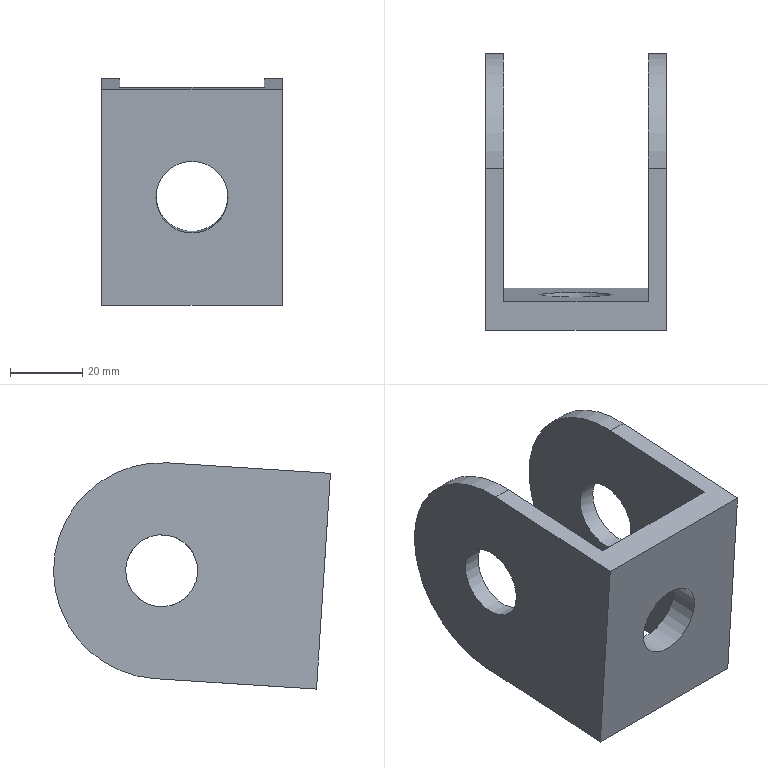Component | NX | CCJ-010 | 1 solid | 13 faces | box 50 x 76.84 x 62.84 mm | volume 54682 mm3 | plane 8 | cylinder 5 | commonest cylinder face diameters 20 x3 60 x2
STEP:
#1=CARTESIAN_POINT('',(0.,0.,0.));
#2=DIRECTION('',(0.,0.,1.));
#3=DIRECTION('',(1.,0.,0.));
#4=AXIS2_PLACEMENT_3D('',#1,#2,#3);
#5=CARTESIAN_POINT('',(5.,79.213,228.609));
#6=VERTEX_POINT('',#5);
#7=CARTESIAN_POINT('',(5.,42.29,226.225));
#8=VERTEX_POINT('',#7);
#9=CARTESIAN_POINT('',(5.,118.132,231.122));
#10=DIRECTION('',(0.,-0.9979,-0.06443));
#11=VECTOR('',#10,1.);
#12=LINE('',#9,#11);
#13=CARTESIAN_POINT('',(0.,109.151,230.542));
#14=DIRECTION('',(0.,0.06443,-0.9979));
#15=DIRECTION('',(-1.,0.,-0.));
#16=AXIS2_PLACEMENT_3D('',#13,#14,#15);
#17=PLANE('',#16);
#18=CARTESIAN_POINT('',(-5.,9.));
#19=DIRECTION('',(0.,-1.));
#20=VECTOR('',#19,1.);
#21=LINE('',#18,#20);
#22=(GEOMETRIC_REPRESENTATION_CONTEXT(2)PARAMETRIC_REPRESENTATION_CONTEXT()REPRESENTATION_CONTEXT('',''));
#23=DEFINITIONAL_REPRESENTATION('',(#21),#22);
#24=PCURVE('',#17,#23);
#25=CARTESIAN_POINT('',(5.,123.287,151.289));
#26=DIRECTION('',(-1.,0.,0.));
#27=DIRECTION('',(0.,0.9979,0.06443));
#28=AXIS2_PLACEMENT_3D('',#25,#26,#27);
#29=PLANE('',#28);
#30=CARTESIAN_POINT('',(-0.,-80.));
#31=DIRECTION('',(-1.,0.));
#32=VECTOR('',#31,1.);
#33=LINE('',#30,#32);
#34=(GEOMETRIC_REPRESENTATION_CONTEXT(2)PARAMETRIC_REPRESENTATION_CONTEXT()REPRESENTATION_CONTEXT('',''));
#35=DEFINITIONAL_REPRESENTATION('',(#33),#34);
#36=PCURVE('',#29,#35);
#37=SURFACE_CURVE('',#12,(#24,#36),.PCURVE_S1.);
#38=EDGE_CURVE('',#6,#8,#37,.T.);
#39=ORIENTED_EDGE('',*,*,#38,.F.);
#40=CARTESIAN_POINT('',(0.,79.213,228.609));
#41=VERTEX_POINT('',#40);
#42=CARTESIAN_POINT('',(0.,79.213,228.609));
#43=DIRECTION('',(-1.,0.,-0.));
#44=VECTOR('',#43,1.);
#45=LINE('',#42,#44);
#46=CARTESIAN_POINT('',(0.,-30.));
#47=DIRECTION('',(1.,0.));
#48=VECTOR('',#47,1.);
#49=LINE('',#46,#48);
#50=(GEOMETRIC_REPRESENTATION_CONTEXT(2)PARAMETRIC_REPRESENTATION_CONTEXT()REPRESENTATION_CONTEXT('',''));
#51=DEFINITIONAL_REPRESENTATION('',(#49),#50);
#52=PCURVE('',#17,#51);
#53=CARTESIAN_POINT('',(0.,81.146,198.672));
#54=DIRECTION('',(-1.,0.,-0.));
#55=DIRECTION('',(-0.,-0.06443,0.9979));
#56=AXIS2_PLACEMENT_3D('',#53,#54,#55);
#57=CYLINDRICAL_SURFACE('',#56,30.);
#58=CARTESIAN_POINT('',(0.,0.));
#59=DIRECTION('',(0.,1.));
#60=VECTOR('',#59,1.);
#61=LINE('',#58,#60);
#62=(GEOMETRIC_REPRESENTATION_CONTEXT(2)PARAMETRIC_REPRESENTATION_CONTEXT()REPRESENTATION_CONTEXT('',''));
#63=DEFINITIONAL_REPRESENTATION('',(#61),#62);
#64=PCURVE('',#57,#63);
#65=SURFACE_CURVE('',#45,(#52,#64),.PCURVE_S1.);
#66=EDGE_CURVE('',#6,#41,#65,.T.);
#67=ORIENTED_EDGE('',*,*,#66,.T.);
#68=CARTESIAN_POINT('',(0.,34.307,225.71));
#69=VERTEX_POINT('',#68);
#70=CARTESIAN_POINT('',(0.,109.151,230.542));
#71=DIRECTION('',(0.,-0.9979,-0.06443));
#72=VECTOR('',#71,1.);
#73=LINE('',#70,#72);
#74=CARTESIAN_POINT('',(0.,0.));
#75=DIRECTION('',(0.,-1.));
#76=VECTOR('',#75,1.);
#77=LINE('',#74,#76);
#78=(GEOMETRIC_REPRESENTATION_CONTEXT(2)PARAMETRIC_REPRESENTATION_CONTEXT()REPRESENTATION_CONTEXT('',''));
#79=DEFINITIONAL_REPRESENTATION('',(#77),#78);
#80=PCURVE('',#17,#79);
#81=CARTESIAN_POINT('',(0.,113.017,170.667));
#82=DIRECTION('',(1.,0.,0.));
#83=DIRECTION('',(0.,-0.9979,-0.06443));
#84=AXIS2_PLACEMENT_3D('',#81,#82,#83);
#85=PLANE('',#84);
#86=CARTESIAN_POINT('',(0.,-60.));
#87=DIRECTION('',(1.,0.));
#88=VECTOR('',#87,1.);
#89=LINE('',#86,#88);
#90=(GEOMETRIC_REPRESENTATION_CONTEXT(2)PARAMETRIC_REPRESENTATION_CONTEXT()REPRESENTATION_CONTEXT('',''));
#91=DEFINITIONAL_REPRESENTATION('',(#89),#90);
#92=PCURVE('',#85,#91);
#93=SURFACE_CURVE('',#73,(#80,#92),.PCURVE_S1.);
#94=EDGE_CURVE('',#41,#69,#93,.T.);
#95=ORIENTED_EDGE('',*,*,#94,.T.);
#96=CARTESIAN_POINT('',(50.,34.307,225.71));
#97=VERTEX_POINT('',#96);
#98=CARTESIAN_POINT('',(0.,34.307,225.71));
#99=DIRECTION('',(1.,-0.,0.));
#100=VECTOR('',#99,1.);
#101=LINE('',#98,#100);
#102=CARTESIAN_POINT('',(0.,-75.));
#103=DIRECTION('',(-1.,-0.));
#104=VECTOR('',#103,1.);
#105=LINE('',#102,#104);
#106=(GEOMETRIC_REPRESENTATION_CONTEXT(2)PARAMETRIC_REPRESENTATION_CONTEXT()REPRESENTATION_CONTEXT('',''));
#107=DEFINITIONAL_REPRESENTATION('',(#105),#106);
#108=PCURVE('',#17,#107);
#109=CARTESIAN_POINT('',(0.,34.307,225.71));
#110=DIRECTION('',(0.,0.9979,0.06443));
#111=DIRECTION('',(1.,0.,0.));
#112=AXIS2_PLACEMENT_3D('',#109,#110,#111);
#113=PLANE('',#112);
#114=CARTESIAN_POINT('',(0.,0.));
#115=DIRECTION('',(1.,-0.));
#116=VECTOR('',#115,1.);
#117=LINE('',#114,#116);
#118=(GEOMETRIC_REPRESENTATION_CONTEXT(2)PARAMETRIC_REPRESENTATION_CONTEXT()REPRESENTATION_CONTEXT('',''));
#119=DEFINITIONAL_REPRESENTATION('',(#117),#118);
#120=PCURVE('',#113,#119);
#121=SURFACE_CURVE('',#101,(#108,#120),.PCURVE_S1.);
#122=EDGE_CURVE('',#69,#97,#121,.T.);
#123=ORIENTED_EDGE('',*,*,#122,.T.);
#124=CARTESIAN_POINT('',(50.,79.213,228.609));
#125=VERTEX_POINT('',#124);
#126=CARTESIAN_POINT('',(50.,109.151,230.542));
#127=DIRECTION('',(0.,-0.9979,-0.06443));
#128=VECTOR('',#127,1.);
#129=LINE('',#126,#128);
#130=CARTESIAN_POINT('',(-50.,-0.));
#131=DIRECTION('',(0.,-1.));
#132=VECTOR('',#131,1.);
#133=LINE('',#130,#132);
#134=(GEOMETRIC_REPRESENTATION_CONTEXT(2)PARAMETRIC_REPRESENTATION_CONTEXT()REPRESENTATION_CONTEXT('',''));
#135=DEFINITIONAL_REPRESENTATION('',(#133),#134);
#136=PCURVE('',#17,#135);
#137=CARTESIAN_POINT('',(50.,109.151,230.542));
#138=DIRECTION('',(-1.,-0.,0.));
#139=DIRECTION('',(0.,-0.06443,0.9979));
#140=AXIS2_PLACEMENT_3D('',#137,#138,#139);
#141=PLANE('',#140);
#142=CARTESIAN_POINT('',(0.,0.));
#143=DIRECTION('',(0.,-1.));
#144=VECTOR('',#143,1.);
#145=LINE('',#142,#144);
#146=(GEOMETRIC_REPRESENTATION_CONTEXT(2)PARAMETRIC_REPRESENTATION_CONTEXT()REPRESENTATION_CONTEXT('',''));
#147=DEFINITIONAL_REPRESENTATION('',(#145),#146);
#148=PCURVE('',#141,#147);
#149=SURFACE_CURVE('',#129,(#136,#148),.PCURVE_S1.);
#150=EDGE_CURVE('',#125,#97,#149,.T.);
#151=ORIENTED_EDGE('',*,*,#150,.F.);
#152=CARTESIAN_POINT('',(45.,79.213,228.609));
#153=VERTEX_POINT('',#152);
#154=CARTESIAN_POINT('',(0.,79.213,228.609));
#155=DIRECTION('',(-1.,0.,-0.));
#156=VECTOR('',#155,1.);
#157=LINE('',#154,#156);
#158=CARTESIAN_POINT('',(0.,-30.));
#159=DIRECTION('',(1.,0.));
#160=VECTOR('',#159,1.);
#161=LINE('',#158,#160);
#162=(GEOMETRIC_REPRESENTATION_CONTEXT(2)PARAMETRIC_REPRESENTATION_CONTEXT()REPRESENTATION_CONTEXT('',''));
#163=DEFINITIONAL_REPRESENTATION('',(#161),#162);
#164=PCURVE('',#17,#163);
#165=CARTESIAN_POINT('',(0.,81.146,198.672));
#166=DIRECTION('',(-1.,0.,-0.));
#167=DIRECTION('',(-0.,-0.06443,0.9979));
#168=AXIS2_PLACEMENT_3D('',#165,#166,#167);
#169=CYLINDRICAL_SURFACE('',#168,30.);
#170=CARTESIAN_POINT('',(0.,0.));
#171=DIRECTION('',(0.,1.));
#172=VECTOR('',#171,1.);
#173=LINE('',#170,#172);
#174=(GEOMETRIC_REPRESENTATION_CONTEXT(2)PARAMETRIC_REPRESENTATION_CONTEXT()REPRESENTATION_CONTEXT('',''));
#175=DEFINITIONAL_REPRESENTATION('',(#173),#174);
#176=PCURVE('',#169,#175);
#177=SURFACE_CURVE('',#157,(#164,#176),.PCURVE_S1.);
#178=EDGE_CURVE('',#125,#153,#177,.T.);
#179=ORIENTED_EDGE('',*,*,#178,.T.);
#180=CARTESIAN_POINT('',(45.,42.29,226.225));
#181=VERTEX_POINT('',#180);
#182=CARTESIAN_POINT('',(45.,42.29,226.225));
#183=DIRECTION('',(0.,0.9979,0.06443));
#184=VECTOR('',#183,1.);
#185=LINE('',#182,#184);
#186=CARTESIAN_POINT('',(-45.,-67.));
#187=DIRECTION('',(-0.,1.));
#188=VECTOR('',#187,1.);
#189=LINE('',#186,#188);
#190=(GEOMETRIC_REPRESENTATION_CONTEXT(2)PARAMETRIC_REPRESENTATION_CONTEXT()REPRESENTATION_CONTEXT('',''));
#191=DEFINITIONAL_REPRESENTATION('',(#189),#190);
#192=PCURVE('',#17,#191);
#193=CARTESIAN_POINT('',(45.,47.445,146.392));
#194=DIRECTION('',(1.,0.,0.));
#195=DIRECTION('',(0.,-0.9979,-0.06443));
#196=AXIS2_PLACEMENT_3D('',#193,#194,#195);
#197=PLANE('',#196);
#198=CARTESIAN_POINT('',(-0.,-80.));
#199=DIRECTION('',(-1.,-0.));
#200=VECTOR('',#199,1.);
#201=LINE('',#198,#200);
#202=(GEOMETRIC_REPRESENTATION_CONTEXT(2)PARAMETRIC_REPRESENTATION_CONTEXT()REPRESENTATION_CONTEXT('',''));
#203=DEFINITIONAL_REPRESENTATION('',(#201),#202);
#204=PCURVE('',#197,#203);
#205=SURFACE_CURVE('',#185,(#192,#204),.PCURVE_S1.);
#206=EDGE_CURVE('',#181,#153,#205,.T.);
#207=ORIENTED_EDGE('',*,*,#206,.F.);
#208=CARTESIAN_POINT('',(5.,42.29,226.225));
#209=DIRECTION('',(1.,0.,0.));
#210=VECTOR('',#209,1.);
#211=LINE('',#208,#210);
#212=CARTESIAN_POINT('',(-5.,-67.));
#213=DIRECTION('',(-1.,-0.));
#214=VECTOR('',#213,1.);
#215=LINE('',#212,#214);
#216=(GEOMETRIC_REPRESENTATION_CONTEXT(2)PARAMETRIC_REPRESENTATION_CONTEXT()REPRESENTATION_CONTEXT('',''));
#217=DEFINITIONAL_REPRESENTATION('',(#215),#216);
#218=PCURVE('',#17,#217);
#219=CARTESIAN_POINT('',(5.,47.445,146.392));
#220=DIRECTION('',(0.,-0.9979,-0.06443));
#221=DIRECTION('',(-1.,0.,0.));
#222=AXIS2_PLACEMENT_3D('',#219,#220,#221);
#223=PLANE('',#222);
#224=CARTESIAN_POINT('',(0.,-80.));
#225=DIRECTION('',(-1.,0.));
#226=VECTOR('',#225,1.);
#227=LINE('',#224,#226);
#228=(GEOMETRIC_REPRESENTATION_CONTEXT(2)PARAMETRIC_REPRESENTATION_CONTEXT()REPRESENTATION_CONTEXT('',''));
#229=DEFINITIONAL_REPRESENTATION('',(#227),#228);
#230=PCURVE('',#223,#229);
#231=SURFACE_CURVE('',#211,(#218,#230),.PCURVE_S1.);
#232=EDGE_CURVE('',#8,#181,#231,.T.);
#233=ORIENTED_EDGE('',*,*,#232,.F.);
#234=EDGE_LOOP('',(#39,#67,#95,#123,#151,#179,#207,#233));
#235=FACE_BOUND('',#234,.T.);
#236=ADVANCED_FACE('',(#235),#17,.F.);
#237=CARTESIAN_POINT('',(5.,83.079,168.734));
#238=VERTEX_POINT('',#237);
#239=CARTESIAN_POINT('',(5.,81.146,198.672));
#240=DIRECTION('',(1.,0.,0.));
#241=DIRECTION('',(0.,0.9979,0.06443));
#242=AXIS2_PLACEMENT_3D('',#239,#240,#241);
#243=CIRCLE('',#242,30.);
#244=CARTESIAN_POINT('',(7.854,-5.));
#245=DIRECTION('',(-1.,-0.));
#246=VECTOR('',#245,1.);
#247=LINE('',#244,#246);
#248=(GEOMETRIC_REPRESENTATION_CONTEXT(2)PARAMETRIC_REPRESENTATION_CONTEXT()REPRESENTATION_CONTEXT('',''));
#249=DEFINITIONAL_REPRESENTATION('',(#247),#248);
#250=PCURVE('',#57,#249);
#251=CARTESIAN_POINT('',(-9.,-50.));
#252=CARTESIAN_POINT('',(-9.,-101.962));
#253=CARTESIAN_POINT('',(-54.,-75.981));
#254=CARTESIAN_POINT('',(-99.,-50.));
#255=CARTESIAN_POINT('',(-54.,-24.019));
#256=CARTESIAN_POINT('',(-9.,1.962));
#257=CARTESIAN_POINT('',(-9.,-50.));
#258=(BOUNDED_CURVE()B_SPLINE_CURVE(2,(#251,#252,#253,#254,#255,#256,#257),.UNSPECIFIED.,.T.,.F.)B_SPLINE_CURVE_WITH_KNOTS((1,2,2,2,2,1),(-2.094,0.,2.094,4.189,6.283,8.378),.UNSPECIFIED.)CURVE()GEOMETRIC_REPRESENTATION_ITEM()RATIONAL_B_SPLINE_CURVE((1.,0.5,1.,0.5,1.,0.5,1.))REPRESENTATION_ITEM(''));
#259=(GEOMETRIC_REPRESENTATION_CONTEXT(2)PARAMETRIC_REPRESENTATION_CONTEXT()REPRESENTATION_CONTEXT('',''));
#260=DEFINITIONAL_REPRESENTATION('',(#258),#259);
#261=PCURVE('',#29,#260);
#262=SURFACE_CURVE('',#243,(#250,#261),.PCURVE_S1.);
#263=EDGE_CURVE('',#238,#6,#262,.T.);
#264=ORIENTED_EDGE('',*,*,#263,.F.);
#265=CARTESIAN_POINT('',(0.,83.079,168.734));
#266=VERTEX_POINT('',#265);
#267=CARTESIAN_POINT('',(50.,83.079,168.734));
#268=DIRECTION('',(1.,0.,0.));
#269=VECTOR('',#268,1.);
#270=LINE('',#267,#269);
#271=CARTESIAN_POINT('',(3.142,-50.));
#272=DIRECTION('',(0.,-1.));
#273=VECTOR('',#272,1.);
#274=LINE('',#271,#273);
#275=(GEOMETRIC_REPRESENTATION_CONTEXT(2)PARAMETRIC_REPRESENTATION_CONTEXT()REPRESENTATION_CONTEXT('',''));
#276=DEFINITIONAL_REPRESENTATION('',(#274),#275);
#277=PCURVE('',#57,#276);
#278=CARTESIAN_POINT('',(50.,113.017,170.667));
#279=DIRECTION('',(0.,-0.06443,0.9979));
#280=DIRECTION('',(0.,-0.9979,-0.06443));
#281=AXIS2_PLACEMENT_3D('',#278,#279,#280);
#282=PLANE('',#281);
#283=CARTESIAN_POINT('',(30.,0.));
#284=DIRECTION('',(0.,1.));
#285=VECTOR('',#284,1.);
#286=LINE('',#283,#285);
#287=(GEOMETRIC_REPRESENTATION_CONTEXT(2)PARAMETRIC_REPRESENTATION_CONTEXT()REPRESENTATION_CONTEXT('',''));
#288=DEFINITIONAL_REPRESENTATION('',(#286),#287);
#289=PCURVE('',#282,#288);
#290=SURFACE_CURVE('',#270,(#277,#289),.PCURVE_S1.);
#291=EDGE_CURVE('',#266,#238,#290,.T.);
#292=ORIENTED_EDGE('',*,*,#291,.F.);
#293=CARTESIAN_POINT('',(0.,81.146,198.672));
#294=DIRECTION('',(-1.,0.,0.));
#295=DIRECTION('',(0.,-0.9979,-0.06443));
#296=AXIS2_PLACEMENT_3D('',#293,#294,#295);
#297=CIRCLE('',#296,30.);
#298=CARTESIAN_POINT('',(-1.571,-0.));
#299=DIRECTION('',(1.,0.));
#300=VECTOR('',#299,1.);
#301=LINE('',#298,#300);
#302=(GEOMETRIC_REPRESENTATION_CONTEXT(2)PARAMETRIC_REPRESENTATION_CONTEXT()REPRESENTATION_CONTEXT('',''));
#303=DEFINITIONAL_REPRESENTATION('',(#301),#302);
#304=PCURVE('',#57,#303);
#305=CARTESIAN_POINT('',(60.,-30.));
#306=CARTESIAN_POINT('',(60.,-81.962));
#307=CARTESIAN_POINT('',(15.,-55.981));
#308=CARTESIAN_POINT('',(-30.,-30.));
#309=CARTESIAN_POINT('',(15.,-4.019));
#310=CARTESIAN_POINT('',(60.,21.962));
#311=CARTESIAN_POINT('',(60.,-30.));
#312=(BOUNDED_CURVE()B_SPLINE_CURVE(2,(#305,#306,#307,#308,#309,#310,#311),.UNSPECIFIED.,.T.,.F.)B_SPLINE_CURVE_WITH_KNOTS((1,2,2,2,2,1),(-2.094,0.,2.094,4.189,6.283,8.378),.UNSPECIFIED.)CURVE()GEOMETRIC_REPRESENTATION_ITEM()RATIONAL_B_SPLINE_CURVE((1.,0.5,1.,0.5,1.,0.5,1.))REPRESENTATION_ITEM(''));
#313=(GEOMETRIC_REPRESENTATION_CONTEXT(2)PARAMETRIC_REPRESENTATION_CONTEXT()REPRESENTATION_CONTEXT('',''));
#314=DEFINITIONAL_REPRESENTATION('',(#312),#313);
#315=PCURVE('',#85,#314);
#316=SURFACE_CURVE('',#297,(#304,#315),.PCURVE_S1.);
#317=EDGE_CURVE('',#41,#266,#316,.T.);
#318=ORIENTED_EDGE('',*,*,#317,.F.);
#319=ORIENTED_EDGE('',*,*,#66,.F.);
#320=EDGE_LOOP('',(#264,#292,#318,#319));
#321=FACE_BOUND('',#320,.T.);
#322=ADVANCED_FACE('',(#321),#57,.T.);
#323=CARTESIAN_POINT('',(5.,71.167,198.027));
#324=VERTEX_POINT('',#323);
#325=CARTESIAN_POINT('',(5.,91.126,199.316));
#326=VERTEX_POINT('',#325);
#327=CARTESIAN_POINT('',(5.,81.146,198.672));
#328=DIRECTION('',(1.,0.,0.));
#329=DIRECTION('',(0.,0.9979,0.06443));
#330=AXIS2_PLACEMENT_3D('',#327,#328,#329);
#331=CIRCLE('',#330,10.);
#332=CARTESIAN_POINT('',(-10.,81.146,198.672));
#333=DIRECTION('',(1.,0.,0.));
#334=DIRECTION('',(0.,-0.9979,-0.06443));
#335=AXIS2_PLACEMENT_3D('',#332,#333,#334);
#336=CYLINDRICAL_SURFACE('',#335,10.);
#337=CARTESIAN_POINT('',(-3.142,15.));
#338=DIRECTION('',(1.,0.));
#339=VECTOR('',#338,1.);
#340=LINE('',#337,#339);
#341=(GEOMETRIC_REPRESENTATION_CONTEXT(2)PARAMETRIC_REPRESENTATION_CONTEXT()REPRESENTATION_CONTEXT('',''));
#342=DEFINITIONAL_REPRESENTATION('',(#340),#341);
#343=PCURVE('',#336,#342);
#344=CARTESIAN_POINT('',(-29.,-50.));
#345=CARTESIAN_POINT('',(-29.,-67.321));
#346=CARTESIAN_POINT('',(-44.,-58.66));
#347=CARTESIAN_POINT('',(-59.,-50.));
#348=CARTESIAN_POINT('',(-44.,-41.34));
#349=CARTESIAN_POINT('',(-29.,-32.679));
#350=CARTESIAN_POINT('',(-29.,-50.));
#351=(BOUNDED_CURVE()B_SPLINE_CURVE(2,(#344,#345,#346,#347,#348,#349,#350),.UNSPECIFIED.,.T.,.F.)B_SPLINE_CURVE_WITH_KNOTS((1,2,2,2,2,1),(-2.094,0.,2.094,4.189,6.283,8.378),.UNSPECIFIED.)CURVE()GEOMETRIC_REPRESENTATION_ITEM()RATIONAL_B_SPLINE_CURVE((1.,0.5,1.,0.5,1.,0.5,1.))REPRESENTATION_ITEM(''));
#352=(GEOMETRIC_REPRESENTATION_CONTEXT(2)PARAMETRIC_REPRESENTATION_CONTEXT()REPRESENTATION_CONTEXT('',''));
#353=DEFINITIONAL_REPRESENTATION('',(#351),#352);
#354=PCURVE('',#29,#353);
#355=SURFACE_CURVE('',#331,(#343,#354),.PCURVE_S1.);
#356=EDGE_CURVE('',#324,#326,#355,.T.);
#357=ORIENTED_EDGE('',*,*,#356,.F.);
#358=CARTESIAN_POINT('',(0.,71.167,198.027));
#359=VERTEX_POINT('',#358);
#360=CARTESIAN_POINT('',(0.,71.167,198.027));
#361=CARTESIAN_POINT('',(5.,71.167,198.027));
#362=B_SPLINE_CURVE_WITH_KNOTS('',1,(#360,#361),.UNSPECIFIED.,.F.,.F.,(2,2),(10.,15.),.PIECEWISE_BEZIER_KNOTS.);
#363=CARTESIAN_POINT('',(0.,0.));
#364=DIRECTION('',(0.,1.));
#365=VECTOR('',#364,1.);
#366=LINE('',#363,#365);
#367=(GEOMETRIC_REPRESENTATION_CONTEXT(2)PARAMETRIC_REPRESENTATION_CONTEXT()REPRESENTATION_CONTEXT('',''));
#368=DEFINITIONAL_REPRESENTATION('',(#366),#367);
#369=PCURVE('',#336,#368);
#370=CARTESIAN_POINT('',(6.283,0.));
#371=DIRECTION('',(0.,1.));
#372=VECTOR('',#371,1.);
#373=LINE('',#370,#372);
#374=(GEOMETRIC_REPRESENTATION_CONTEXT(2)PARAMETRIC_REPRESENTATION_CONTEXT()REPRESENTATION_CONTEXT('',''));
#375=DEFINITIONAL_REPRESENTATION('',(#373),#374);
#376=PCURVE('',#336,#375);
#377=SEAM_CURVE('',#362,(#369,#376),.PCURVE_S1.);
#378=EDGE_CURVE('',#359,#324,#377,.T.);
#379=ORIENTED_EDGE('',*,*,#378,.F.);
#380=CARTESIAN_POINT('',(0.,81.146,198.672));
#381=DIRECTION('',(1.,0.,0.));
#382=DIRECTION('',(0.,-0.9979,-0.06443));
#383=AXIS2_PLACEMENT_3D('',#380,#381,#382);
#384=CIRCLE('',#383,10.);
#385=CARTESIAN_POINT('',(0.,10.));
#386=DIRECTION('',(1.,0.));
#387=VECTOR('',#386,1.);
#388=LINE('',#385,#387);
#389=(GEOMETRIC_REPRESENTATION_CONTEXT(2)PARAMETRIC_REPRESENTATION_CONTEXT()REPRESENTATION_CONTEXT('',''));
#390=DEFINITIONAL_REPRESENTATION('',(#388),#389);
#391=PCURVE('',#336,#390);
#392=CARTESIAN_POINT('',(30.,-30.));
#393=DIRECTION('',(1.,0.));
#394=AXIS2_PLACEMENT_2D('',#392,#393);
#395=CIRCLE('',#394,10.);
#396=(GEOMETRIC_REPRESENTATION_CONTEXT(2)PARAMETRIC_REPRESENTATION_CONTEXT()REPRESENTATION_CONTEXT('',''));
#397=DEFINITIONAL_REPRESENTATION('',(#395),#396);
#398=PCURVE('',#85,#397);
#399=SURFACE_CURVE('',#384,(#391,#398),.PCURVE_S1.);
#400=EDGE_CURVE('',#359,#359,#399,.T.);
#401=ORIENTED_EDGE('',*,*,#400,.T.);
#402=ORIENTED_EDGE('',*,*,#378,.T.);
#403=CARTESIAN_POINT('',(5.,81.146,198.672));
#404=DIRECTION('',(1.,0.,0.));
#405=DIRECTION('',(0.,0.9979,0.06443));
#406=AXIS2_PLACEMENT_3D('',#403,#404,#405);
#407=CIRCLE('',#406,10.);
#408=CARTESIAN_POINT('',(3.142,15.));
#409=DIRECTION('',(1.,0.));
#410=VECTOR('',#409,1.);
#411=LINE('',#408,#410);
#412=(GEOMETRIC_REPRESENTATION_CONTEXT(2)PARAMETRIC_REPRESENTATION_CONTEXT()REPRESENTATION_CONTEXT('',''));
#413=DEFINITIONAL_REPRESENTATION('',(#411),#412);
#414=PCURVE('',#336,#413);
#415=CARTESIAN_POINT('',(-29.,-50.));
#416=CARTESIAN_POINT('',(-29.,-67.321));
#417=CARTESIAN_POINT('',(-44.,-58.66));
#418=CARTESIAN_POINT('',(-59.,-50.));
#419=CARTESIAN_POINT('',(-44.,-41.34));
#420=CARTESIAN_POINT('',(-29.,-32.679));
#421=CARTESIAN_POINT('',(-29.,-50.));
#422=(BOUNDED_CURVE()B_SPLINE_CURVE(2,(#415,#416,#417,#418,#419,#420,#421),.UNSPECIFIED.,.T.,.F.)B_SPLINE_CURVE_WITH_KNOTS((1,2,2,2,2,1),(-2.094,0.,2.094,4.189,6.283,8.378),.UNSPECIFIED.)CURVE()GEOMETRIC_REPRESENTATION_ITEM()RATIONAL_B_SPLINE_CURVE((1.,0.5,1.,0.5,1.,0.5,1.))REPRESENTATION_ITEM(''));
#423=(GEOMETRIC_REPRESENTATION_CONTEXT(2)PARAMETRIC_REPRESENTATION_CONTEXT()REPRESENTATION_CONTEXT('',''));
#424=DEFINITIONAL_REPRESENTATION('',(#422),#423);
#425=PCURVE('',#29,#424);
#426=SURFACE_CURVE('',#407,(#414,#425),.PCURVE_S1.);
#427=EDGE_CURVE('',#326,#324,#426,.T.);
#428=ORIENTED_EDGE('',*,*,#427,.F.);
#429=EDGE_LOOP('',(#357,#379,#401,#402,#428));
#430=FACE_BOUND('',#429,.F.);
#431=ADVANCED_FACE('',(#430),#336,.F.);
#432=CARTESIAN_POINT('',(45.,71.167,198.027));
#433=VERTEX_POINT('',#432);
#434=CARTESIAN_POINT('',(45.,81.146,198.672));
#435=DIRECTION('',(-1.,0.,0.));
#436=DIRECTION('',(0.,-0.9979,-0.06443));
#437=AXIS2_PLACEMENT_3D('',#434,#435,#436);
#438=CIRCLE('',#437,10.);
#439=CARTESIAN_POINT('',(-10.,81.146,198.672));
#440=DIRECTION('',(1.,0.,0.));
#441=DIRECTION('',(0.,-0.9979,-0.06443));
#442=AXIS2_PLACEMENT_3D('',#439,#440,#441);
#443=CYLINDRICAL_SURFACE('',#442,10.);
#444=CARTESIAN_POINT('',(6.283,55.));
#445=DIRECTION('',(-1.,0.));
#446=VECTOR('',#445,1.);
#447=LINE('',#444,#446);
#448=(GEOMETRIC_REPRESENTATION_CONTEXT(2)PARAMETRIC_REPRESENTATION_CONTEXT()REPRESENTATION_CONTEXT('',''));
#449=DEFINITIONAL_REPRESENTATION('',(#447),#448);
#450=PCURVE('',#443,#449);
#451=CARTESIAN_POINT('',(-27.,-50.));
#452=CARTESIAN_POINT('',(-27.,-67.321));
#453=CARTESIAN_POINT('',(-42.,-58.66));
#454=CARTESIAN_POINT('',(-57.,-50.));
#455=CARTESIAN_POINT('',(-42.,-41.34));
#456=CARTESIAN_POINT('',(-27.,-32.679));
#457=CARTESIAN_POINT('',(-27.,-50.));
#458=(BOUNDED_CURVE()B_SPLINE_CURVE(2,(#451,#452,#453,#454,#455,#456,#457),.UNSPECIFIED.,.T.,.F.)B_SPLINE_CURVE_WITH_KNOTS((1,2,2,2,2,1),(-2.094,0.,2.094,4.189,6.283,8.378),.UNSPECIFIED.)CURVE()GEOMETRIC_REPRESENTATION_ITEM()RATIONAL_B_SPLINE_CURVE((1.,0.5,1.,0.5,1.,0.5,1.))REPRESENTATION_ITEM(''));
#459=(GEOMETRIC_REPRESENTATION_CONTEXT(2)PARAMETRIC_REPRESENTATION_CONTEXT()REPRESENTATION_CONTEXT('',''));
#460=DEFINITIONAL_REPRESENTATION('',(#458),#459);
#461=PCURVE('',#197,#460);
#462=SURFACE_CURVE('',#438,(#450,#461),.PCURVE_S1.);
#463=EDGE_CURVE('',#433,#433,#462,.T.);
#464=ORIENTED_EDGE('',*,*,#463,.F.);
#465=CARTESIAN_POINT('',(50.,71.167,198.027));
#466=VERTEX_POINT('',#465);
#467=CARTESIAN_POINT('',(45.,71.167,198.027));
#468=CARTESIAN_POINT('',(50.,71.167,198.027));
#469=B_SPLINE_CURVE_WITH_KNOTS('',1,(#467,#468),.UNSPECIFIED.,.F.,.F.,(2,2),(55.,60.),.PIECEWISE_BEZIER_KNOTS.);
#470=CARTESIAN_POINT('',(6.283,0.));
#471=DIRECTION('',(0.,1.));
#472=VECTOR('',#471,1.);
#473=LINE('',#470,#472);
#474=(GEOMETRIC_REPRESENTATION_CONTEXT(2)PARAMETRIC_REPRESENTATION_CONTEXT()REPRESENTATION_CONTEXT('',''));
#475=DEFINITIONAL_REPRESENTATION('',(#473),#474);
#476=PCURVE('',#443,#475);
#477=CARTESIAN_POINT('',(0.,0.));
#478=DIRECTION('',(0.,1.));
#479=VECTOR('',#478,1.);
#480=LINE('',#477,#479);
#481=(GEOMETRIC_REPRESENTATION_CONTEXT(2)PARAMETRIC_REPRESENTATION_CONTEXT()REPRESENTATION_CONTEXT('',''));
#482=DEFINITIONAL_REPRESENTATION('',(#480),#481);
#483=PCURVE('',#443,#482);
#484=SEAM_CURVE('',#469,(#476,#483),.PCURVE_S1.);
#485=EDGE_CURVE('',#433,#466,#484,.T.);
#486=ORIENTED_EDGE('',*,*,#485,.T.);
#487=CARTESIAN_POINT('',(50.,81.791,188.693));
#488=VERTEX_POINT('',#487);
#489=CARTESIAN_POINT('',(50.,81.146,198.672));
#490=DIRECTION('',(1.,0.,0.));
#491=DIRECTION('',(0.,0.06443,-0.9979));
#492=AXIS2_PLACEMENT_3D('',#489,#490,#491);
#493=CIRCLE('',#492,10.);
#494=CARTESIAN_POINT('',(1.571,60.));
#495=DIRECTION('',(1.,0.));
#496=VECTOR('',#495,1.);
#497=LINE('',#494,#496);
#498=(GEOMETRIC_REPRESENTATION_CONTEXT(2)PARAMETRIC_REPRESENTATION_CONTEXT()REPRESENTATION_CONTEXT('',''));
#499=DEFINITIONAL_REPRESENTATION('',(#497),#498);
#500=PCURVE('',#443,#499);
#501=CARTESIAN_POINT('',(-40.,-30.));
#502=CARTESIAN_POINT('',(-40.,-12.679));
#503=CARTESIAN_POINT('',(-25.,-21.34));
#504=CARTESIAN_POINT('',(-10.,-30.));
#505=CARTESIAN_POINT('',(-25.,-38.66));
#506=CARTESIAN_POINT('',(-40.,-47.321));
#507=CARTESIAN_POINT('',(-40.,-30.));
#508=(BOUNDED_CURVE()B_SPLINE_CURVE(2,(#501,#502,#503,#504,#505,#506,#507),.UNSPECIFIED.,.T.,.F.)B_SPLINE_CURVE_WITH_KNOTS((1,2,2,2,2,1),(-2.094,0.,2.094,4.189,6.283,8.378),.UNSPECIFIED.)CURVE()GEOMETRIC_REPRESENTATION_ITEM()RATIONAL_B_SPLINE_CURVE((1.,0.5,1.,0.5,1.,0.5,1.))REPRESENTATION_ITEM(''));
#509=(GEOMETRIC_REPRESENTATION_CONTEXT(2)PARAMETRIC_REPRESENTATION_CONTEXT()REPRESENTATION_CONTEXT('',''));
#510=DEFINITIONAL_REPRESENTATION('',(#508),#509);
#511=PCURVE('',#141,#510);
#512=SURFACE_CURVE('',#493,(#500,#511),.PCURVE_S1.);
#513=EDGE_CURVE('',#488,#466,#512,.T.);
#514=ORIENTED_EDGE('',*,*,#513,.F.);
#515=CARTESIAN_POINT('',(50.,81.146,198.672));
#516=DIRECTION('',(1.,0.,0.));
#517=DIRECTION('',(0.,0.06443,-0.9979));
#518=AXIS2_PLACEMENT_3D('',#515,#516,#517);
#519=CIRCLE('',#518,10.);
#520=CARTESIAN_POINT('',(-4.712,60.));
#521=DIRECTION('',(1.,0.));
#522=VECTOR('',#521,1.);
#523=LINE('',#520,#522);
#524=(GEOMETRIC_REPRESENTATION_CONTEXT(2)PARAMETRIC_REPRESENTATION_CONTEXT()REPRESENTATION_CONTEXT('',''));
#525=DEFINITIONAL_REPRESENTATION('',(#523),#524);
#526=PCURVE('',#443,#525);
#527=CARTESIAN_POINT('',(-40.,-30.));
#528=CARTESIAN_POINT('',(-40.,-12.679));
#529=CARTESIAN_POINT('',(-25.,-21.34));
#530=CARTESIAN_POINT('',(-10.,-30.));
#531=CARTESIAN_POINT('',(-25.,-38.66));
#532=CARTESIAN_POINT('',(-40.,-47.321));
#533=CARTESIAN_POINT('',(-40.,-30.));
#534=(BOUNDED_CURVE()B_SPLINE_CURVE(2,(#527,#528,#529,#530,#531,#532,#533),.UNSPECIFIED.,.T.,.F.)B_SPLINE_CURVE_WITH_KNOTS((1,2,2,2,2,1),(-2.094,0.,2.094,4.189,6.283,8.378),.UNSPECIFIED.)CURVE()GEOMETRIC_REPRESENTATION_ITEM()RATIONAL_B_SPLINE_CURVE((1.,0.5,1.,0.5,1.,0.5,1.))REPRESENTATION_ITEM(''));
#535=(GEOMETRIC_REPRESENTATION_CONTEXT(2)PARAMETRIC_REPRESENTATION_CONTEXT()REPRESENTATION_CONTEXT('',''));
#536=DEFINITIONAL_REPRESENTATION('',(#534),#535);
#537=PCURVE('',#141,#536);
#538=SURFACE_CURVE('',#519,(#526,#537),.PCURVE_S1.);
#539=EDGE_CURVE('',#466,#488,#538,.T.);
#540=ORIENTED_EDGE('',*,*,#539,.F.);
#541=ORIENTED_EDGE('',*,*,#485,.F.);
#542=EDGE_LOOP('',(#464,#486,#514,#540,#541));
#543=FACE_BOUND('',#542,.F.);
#544=ADVANCED_FACE('',(#543),#443,.F.);
#545=CARTESIAN_POINT('',(50.,83.079,168.734));
#546=VERTEX_POINT('',#545);
#547=CARTESIAN_POINT('',(50.,38.173,165.835));
#548=VERTEX_POINT('',#547);
#549=CARTESIAN_POINT('',(50.,113.017,170.667));
#550=DIRECTION('',(0.,-0.9979,-0.06443));
#551=VECTOR('',#550,1.);
#552=LINE('',#549,#551);
#553=CARTESIAN_POINT('',(-60.,0.));
#554=DIRECTION('',(0.,-1.));
#555=VECTOR('',#554,1.);
#556=LINE('',#553,#555);
#557=(GEOMETRIC_REPRESENTATION_CONTEXT(2)PARAMETRIC_REPRESENTATION_CONTEXT()REPRESENTATION_CONTEXT('',''));
#558=DEFINITIONAL_REPRESENTATION('',(#556),#557);
#559=PCURVE('',#141,#558);
#560=CARTESIAN_POINT('',(0.,0.));
#561=DIRECTION('',(1.,0.));
#562=VECTOR('',#561,1.);
#563=LINE('',#560,#562);
#564=(GEOMETRIC_REPRESENTATION_CONTEXT(2)PARAMETRIC_REPRESENTATION_CONTEXT()REPRESENTATION_CONTEXT('',''));
#565=DEFINITIONAL_REPRESENTATION('',(#563),#564);
#566=PCURVE('',#282,#565);
#567=SURFACE_CURVE('',#552,(#559,#566),.PCURVE_S1.);
#568=EDGE_CURVE('',#546,#548,#567,.T.);
#569=ORIENTED_EDGE('',*,*,#568,.F.);
#570=CARTESIAN_POINT('',(50.,81.146,198.672));
#571=DIRECTION('',(1.,0.,-0.));
#572=DIRECTION('',(0.,-0.06443,0.9979));
#573=AXIS2_PLACEMENT_3D('',#570,#571,#572);
#574=CIRCLE('',#573,30.);
#575=CARTESIAN_POINT('',(0.,-30.));
#576=CARTESIAN_POINT('',(0.,-81.962));
#577=CARTESIAN_POINT('',(-45.,-55.981));
#578=CARTESIAN_POINT('',(-90.,-30.));
#579=CARTESIAN_POINT('',(-45.,-4.019));
#580=CARTESIAN_POINT('',(0.,21.962));
#581=CARTESIAN_POINT('',(0.,-30.));
#582=(BOUNDED_CURVE()B_SPLINE_CURVE(2,(#575,#576,#577,#578,#579,#580,#581),.UNSPECIFIED.,.T.,.F.)B_SPLINE_CURVE_WITH_KNOTS((1,2,2,2,2,1),(-2.094,0.,2.094,4.189,6.283,8.378),.UNSPECIFIED.)CURVE()GEOMETRIC_REPRESENTATION_ITEM()RATIONAL_B_SPLINE_CURVE((1.,0.5,1.,0.5,1.,0.5,1.))REPRESENTATION_ITEM(''));
#583=(GEOMETRIC_REPRESENTATION_CONTEXT(2)PARAMETRIC_REPRESENTATION_CONTEXT()REPRESENTATION_CONTEXT('',''));
#584=DEFINITIONAL_REPRESENTATION('',(#582),#583);
#585=PCURVE('',#141,#584);
#586=CARTESIAN_POINT('',(6.283,-50.));
#587=DIRECTION('',(-1.,-0.));
#588=VECTOR('',#587,1.);
#589=LINE('',#586,#588);
#590=(GEOMETRIC_REPRESENTATION_CONTEXT(2)PARAMETRIC_REPRESENTATION_CONTEXT()REPRESENTATION_CONTEXT('',''));
#591=DEFINITIONAL_REPRESENTATION('',(#589),#590);
#592=PCURVE('',#169,#591);
#593=SURFACE_CURVE('',#574,(#585,#592),.PCURVE_S1.);
#594=EDGE_CURVE('',#546,#125,#593,.T.);
#595=ORIENTED_EDGE('',*,*,#594,.T.);
#596=ORIENTED_EDGE('',*,*,#150,.T.);
#597=CARTESIAN_POINT('',(50.,34.307,225.71));
#598=DIRECTION('',(-0.,0.06443,-0.9979));
#599=VECTOR('',#598,1.);
#600=LINE('',#597,#599);
#601=CARTESIAN_POINT('',(0.,-75.));
#602=DIRECTION('',(-1.,0.));
#603=VECTOR('',#602,1.);
#604=LINE('',#601,#603);
#605=(GEOMETRIC_REPRESENTATION_CONTEXT(2)PARAMETRIC_REPRESENTATION_CONTEXT()REPRESENTATION_CONTEXT('',''));
#606=DEFINITIONAL_REPRESENTATION('',(#604),#605);
#607=PCURVE('',#141,#606);
#608=CARTESIAN_POINT('',(50.,0.));
#609=DIRECTION('',(-0.,1.));
#610=VECTOR('',#609,1.);
#611=LINE('',#608,#610);
#612=(GEOMETRIC_REPRESENTATION_CONTEXT(2)PARAMETRIC_REPRESENTATION_CONTEXT()REPRESENTATION_CONTEXT('',''));
#613=DEFINITIONAL_REPRESENTATION('',(#611),#612);
#614=PCURVE('',#113,#613);
#615=SURFACE_CURVE('',#600,(#607,#614),.PCURVE_S1.);
#616=EDGE_CURVE('',#97,#548,#615,.T.);
#617=ORIENTED_EDGE('',*,*,#616,.T.);
#618=EDGE_LOOP('',(#569,#595,#596,#617));
#619=FACE_BOUND('',#618,.T.);
#620=ORIENTED_EDGE('',*,*,#513,.F.);
#621=ORIENTED_EDGE('',*,*,#539,.F.);
#622=EDGE_LOOP('',(#620,#621));
#623=FACE_BOUND('',#622,.T.);
#624=ADVANCED_FACE('',(#619,#623),#141,.F.);
#625=ORIENTED_EDGE('',*,*,#400,.T.);
#626=EDGE_LOOP('',(#625));
#627=FACE_BOUND('',#626,.T.);
#628=ORIENTED_EDGE('',*,*,#317,.T.);
#629=CARTESIAN_POINT('',(0.,38.173,165.835));
#630=VERTEX_POINT('',#629);
#631=CARTESIAN_POINT('',(0.,113.017,170.667));
#632=DIRECTION('',(0.,-0.9979,-0.06443));
#633=VECTOR('',#632,1.);
#634=LINE('',#631,#633);
#635=CARTESIAN_POINT('',(0.,0.));
#636=DIRECTION('',(1.,0.));
#637=VECTOR('',#636,1.);
#638=LINE('',#635,#637);
#639=(GEOMETRIC_REPRESENTATION_CONTEXT(2)PARAMETRIC_REPRESENTATION_CONTEXT()REPRESENTATION_CONTEXT('',''));
#640=DEFINITIONAL_REPRESENTATION('',(#638),#639);
#641=PCURVE('',#85,#640);
#642=CARTESIAN_POINT('',(0.,-50.));
#643=DIRECTION('',(1.,0.));
#644=VECTOR('',#643,1.);
#645=LINE('',#642,#644);
#646=(GEOMETRIC_REPRESENTATION_CONTEXT(2)PARAMETRIC_REPRESENTATION_CONTEXT()REPRESENTATION_CONTEXT('',''));
#647=DEFINITIONAL_REPRESENTATION('',(#645),#646);
#648=PCURVE('',#282,#647);
#649=SURFACE_CURVE('',#634,(#641,#648),.PCURVE_S1.);
#650=EDGE_CURVE('',#266,#630,#649,.T.);
#651=ORIENTED_EDGE('',*,*,#650,.T.);
#652=CARTESIAN_POINT('',(0.,38.173,165.835));
#653=DIRECTION('',(0.,-0.06443,0.9979));
#654=VECTOR('',#653,1.);
#655=LINE('',#652,#654);
#656=CARTESIAN_POINT('',(75.,-0.));
#657=DIRECTION('',(0.,-1.));
#658=VECTOR('',#657,1.);
#659=LINE('',#656,#658);
#660=(GEOMETRIC_REPRESENTATION_CONTEXT(2)PARAMETRIC_REPRESENTATION_CONTEXT()REPRESENTATION_CONTEXT('',''));
#661=DEFINITIONAL_REPRESENTATION('',(#659),#660);
#662=PCURVE('',#85,#661);
#663=CARTESIAN_POINT('',(0.,60.));
#664=DIRECTION('',(0.,-1.));
#665=VECTOR('',#664,1.);
#666=LINE('',#663,#665);
#667=(GEOMETRIC_REPRESENTATION_CONTEXT(2)PARAMETRIC_REPRESENTATION_CONTEXT()REPRESENTATION_CONTEXT('',''));
#668=DEFINITIONAL_REPRESENTATION('',(#666),#667);
#669=PCURVE('',#113,#668);
#670=SURFACE_CURVE('',#655,(#662,#669),.PCURVE_S1.);
#671=EDGE_CURVE('',#630,#69,#670,.T.);
#672=ORIENTED_EDGE('',*,*,#671,.T.);
#673=ORIENTED_EDGE('',*,*,#94,.F.);
#674=EDGE_LOOP('',(#628,#651,#672,#673));
#675=FACE_BOUND('',#674,.T.);
#676=ADVANCED_FACE('',(#627,#675),#85,.F.);
#677=ORIENTED_EDGE('',*,*,#291,.T.);
#678=CARTESIAN_POINT('',(5.,46.156,166.35));
#679=VERTEX_POINT('',#678);
#680=CARTESIAN_POINT('',(5.,113.017,170.667));
#681=DIRECTION('',(0.,-0.9979,-0.06443));
#682=VECTOR('',#681,1.);
#683=LINE('',#680,#682);
#684=CARTESIAN_POINT('',(0.,-45.));
#685=DIRECTION('',(1.,0.));
#686=VECTOR('',#685,1.);
#687=LINE('',#684,#686);
#688=(GEOMETRIC_REPRESENTATION_CONTEXT(2)PARAMETRIC_REPRESENTATION_CONTEXT()REPRESENTATION_CONTEXT('',''));
#689=DEFINITIONAL_REPRESENTATION('',(#687),#688);
#690=PCURVE('',#282,#689);
#691=CARTESIAN_POINT('',(-9.,-20.));
#692=DIRECTION('',(-1.,0.));
#693=VECTOR('',#692,1.);
#694=LINE('',#691,#693);
#695=(GEOMETRIC_REPRESENTATION_CONTEXT(2)PARAMETRIC_REPRESENTATION_CONTEXT()REPRESENTATION_CONTEXT('',''));
#696=DEFINITIONAL_REPRESENTATION('',(#694),#695);
#697=PCURVE('',#29,#696);
#698=SURFACE_CURVE('',#683,(#690,#697),.PCURVE_S1.);
#699=EDGE_CURVE('',#238,#679,#698,.T.);
#700=ORIENTED_EDGE('',*,*,#699,.T.);
#701=CARTESIAN_POINT('',(45.,46.156,166.35));
#702=VERTEX_POINT('',#701);
#703=CARTESIAN_POINT('',(50.,46.156,166.35));
#704=DIRECTION('',(1.,0.,0.));
#705=VECTOR('',#704,1.);
#706=LINE('',#703,#705);
#707=CARTESIAN_POINT('',(67.,0.));
#708=DIRECTION('',(0.,1.));
#709=VECTOR('',#708,1.);
#710=LINE('',#707,#709);
#711=(GEOMETRIC_REPRESENTATION_CONTEXT(2)PARAMETRIC_REPRESENTATION_CONTEXT()REPRESENTATION_CONTEXT('',''));
#712=DEFINITIONAL_REPRESENTATION('',(#710),#711);
#713=PCURVE('',#282,#712);
#714=CARTESIAN_POINT('',(-45.,-20.));
#715=DIRECTION('',(-1.,0.));
#716=VECTOR('',#715,1.);
#717=LINE('',#714,#716);
#718=(GEOMETRIC_REPRESENTATION_CONTEXT(2)PARAMETRIC_REPRESENTATION_CONTEXT()REPRESENTATION_CONTEXT('',''));
#719=DEFINITIONAL_REPRESENTATION('',(#717),#718);
#720=PCURVE('',#223,#719);
#721=SURFACE_CURVE('',#706,(#713,#720),.PCURVE_S1.);
#722=EDGE_CURVE('',#679,#702,#721,.T.);
#723=ORIENTED_EDGE('',*,*,#722,.T.);
#724=CARTESIAN_POINT('',(45.,83.079,168.734));
#725=VERTEX_POINT('',#724);
#726=CARTESIAN_POINT('',(45.,113.017,170.667));
#727=DIRECTION('',(0.,0.9979,0.06443));
#728=VECTOR('',#727,1.);
#729=LINE('',#726,#728);
#730=CARTESIAN_POINT('',(0.,-5.));
#731=DIRECTION('',(-1.,0.));
#732=VECTOR('',#731,1.);
#733=LINE('',#730,#732);
#734=(GEOMETRIC_REPRESENTATION_CONTEXT(2)PARAMETRIC_REPRESENTATION_CONTEXT()REPRESENTATION_CONTEXT('',''));
#735=DEFINITIONAL_REPRESENTATION('',(#733),#734);
#736=PCURVE('',#282,#735);
#737=CARTESIAN_POINT('',(-67.,-20.));
#738=DIRECTION('',(-1.,0.));
#739=VECTOR('',#738,1.);
#740=LINE('',#737,#739);
#741=(GEOMETRIC_REPRESENTATION_CONTEXT(2)PARAMETRIC_REPRESENTATION_CONTEXT()REPRESENTATION_CONTEXT('',''));
#742=DEFINITIONAL_REPRESENTATION('',(#740),#741);
#743=PCURVE('',#197,#742);
#744=SURFACE_CURVE('',#729,(#736,#743),.PCURVE_S1.);
#745=EDGE_CURVE('',#702,#725,#744,.T.);
#746=ORIENTED_EDGE('',*,*,#745,.T.);
#747=CARTESIAN_POINT('',(50.,83.079,168.734));
#748=DIRECTION('',(1.,0.,0.));
#749=VECTOR('',#748,1.);
#750=LINE('',#747,#749);
#751=CARTESIAN_POINT('',(30.,0.));
#752=DIRECTION('',(0.,1.));
#753=VECTOR('',#752,1.);
#754=LINE('',#751,#753);
#755=(GEOMETRIC_REPRESENTATION_CONTEXT(2)PARAMETRIC_REPRESENTATION_CONTEXT()REPRESENTATION_CONTEXT('',''));
#756=DEFINITIONAL_REPRESENTATION('',(#754),#755);
#757=PCURVE('',#282,#756);
#758=CARTESIAN_POINT('',(3.142,-50.));
#759=DIRECTION('',(0.,-1.));
#760=VECTOR('',#759,1.);
#761=LINE('',#758,#760);
#762=(GEOMETRIC_REPRESENTATION_CONTEXT(2)PARAMETRIC_REPRESENTATION_CONTEXT()REPRESENTATION_CONTEXT('',''));
#763=DEFINITIONAL_REPRESENTATION('',(#761),#762);
#764=PCURVE('',#169,#763);
#765=SURFACE_CURVE('',#750,(#757,#764),.PCURVE_S1.);
#766=EDGE_CURVE('',#725,#546,#765,.T.);
#767=ORIENTED_EDGE('',*,*,#766,.T.);
#768=ORIENTED_EDGE('',*,*,#568,.T.);
#769=CARTESIAN_POINT('',(50.,38.173,165.835));
#770=DIRECTION('',(-1.,0.,0.));
#771=VECTOR('',#770,1.);
#772=LINE('',#769,#771);
#773=CARTESIAN_POINT('',(75.,0.));
#774=DIRECTION('',(0.,-1.));
#775=VECTOR('',#774,1.);
#776=LINE('',#773,#775);
#777=(GEOMETRIC_REPRESENTATION_CONTEXT(2)PARAMETRIC_REPRESENTATION_CONTEXT()REPRESENTATION_CONTEXT('',''));
#778=DEFINITIONAL_REPRESENTATION('',(#776),#777);
#779=PCURVE('',#282,#778);
#780=CARTESIAN_POINT('',(50.,60.));
#781=DIRECTION('',(-1.,0.));
#782=VECTOR('',#781,1.);
#783=LINE('',#780,#782);
#784=(GEOMETRIC_REPRESENTATION_CONTEXT(2)PARAMETRIC_REPRESENTATION_CONTEXT()REPRESENTATION_CONTEXT('',''));
#785=DEFINITIONAL_REPRESENTATION('',(#783),#784);
#786=PCURVE('',#113,#785);
#787=SURFACE_CURVE('',#772,(#779,#786),.PCURVE_S1.);
#788=EDGE_CURVE('',#548,#630,#787,.T.);
#789=ORIENTED_EDGE('',*,*,#788,.T.);
#790=ORIENTED_EDGE('',*,*,#650,.F.);
#791=EDGE_LOOP('',(#677,#700,#723,#746,#767,#768,#789,#790));
#792=FACE_BOUND('',#791,.T.);
#793=ADVANCED_FACE('',(#792),#282,.F.);
#794=CARTESIAN_POINT('',(35.,36.24,195.772));
#795=VERTEX_POINT('',#794);
#796=CARTESIAN_POINT('',(15.,36.24,195.772));
#797=VERTEX_POINT('',#796);
#798=CARTESIAN_POINT('',(25.,36.24,195.772));
#799=DIRECTION('',(0.,0.9979,0.06443));
#800=DIRECTION('',(1.,0.,0.));
#801=AXIS2_PLACEMENT_3D('',#798,#799,#800);
#802=CIRCLE('',#801,10.);
#803=CARTESIAN_POINT('',(25.,30.));
#804=DIRECTION('',(1.,0.));
#805=AXIS2_PLACEMENT_2D('',#803,#804);
#806=CIRCLE('',#805,10.);
#807=(GEOMETRIC_REPRESENTATION_CONTEXT(2)PARAMETRIC_REPRESENTATION_CONTEXT()REPRESENTATION_CONTEXT('',''));
#808=DEFINITIONAL_REPRESENTATION('',(#806),#807);
#809=PCURVE('',#113,#808);
#810=CARTESIAN_POINT('',(25.,96.115,199.638));
#811=DIRECTION('',(0.,-0.9979,-0.06443));
#812=DIRECTION('',(-1.,0.,0.));
#813=AXIS2_PLACEMENT_3D('',#810,#811,#812);
#814=CYLINDRICAL_SURFACE('',#813,10.);
#815=CARTESIAN_POINT('',(3.142,60.));
#816=DIRECTION('',(-1.,0.));
#817=VECTOR('',#816,1.);
#818=LINE('',#815,#817);
#819=(GEOMETRIC_REPRESENTATION_CONTEXT(2)PARAMETRIC_REPRESENTATION_CONTEXT()REPRESENTATION_CONTEXT('',''));
#820=DEFINITIONAL_REPRESENTATION('',(#818),#819);
#821=PCURVE('',#814,#820);
#822=SURFACE_CURVE('',#802,(#809,#821),.PCURVE_S1.);
#823=EDGE_CURVE('',#795,#797,#822,.T.);
#824=ORIENTED_EDGE('',*,*,#823,.T.);
#825=CARTESIAN_POINT('',(25.,36.24,195.772));
#826=DIRECTION('',(0.,0.9979,0.06443));
#827=DIRECTION('',(1.,0.,0.));
#828=AXIS2_PLACEMENT_3D('',#825,#826,#827);
#829=CIRCLE('',#828,10.);
#830=CARTESIAN_POINT('',(25.,30.));
#831=DIRECTION('',(1.,0.));
#832=AXIS2_PLACEMENT_2D('',#830,#831);
#833=CIRCLE('',#832,10.);
#834=(GEOMETRIC_REPRESENTATION_CONTEXT(2)PARAMETRIC_REPRESENTATION_CONTEXT()REPRESENTATION_CONTEXT('',''));
#835=DEFINITIONAL_REPRESENTATION('',(#833),#834);
#836=PCURVE('',#113,#835);
#837=CARTESIAN_POINT('',(9.425,60.));
#838=DIRECTION('',(-1.,0.));
#839=VECTOR('',#838,1.);
#840=LINE('',#837,#839);
#841=(GEOMETRIC_REPRESENTATION_CONTEXT(2)PARAMETRIC_REPRESENTATION_CONTEXT()REPRESENTATION_CONTEXT('',''));
#842=DEFINITIONAL_REPRESENTATION('',(#840),#841);
#843=PCURVE('',#814,#842);
#844=SURFACE_CURVE('',#829,(#836,#843),.PCURVE_S1.);
#845=EDGE_CURVE('',#797,#795,#844,.T.);
#846=ORIENTED_EDGE('',*,*,#845,.T.);
#847=EDGE_LOOP('',(#824,#846));
#848=FACE_BOUND('',#847,.T.);
#849=ORIENTED_EDGE('',*,*,#671,.F.);
#850=ORIENTED_EDGE('',*,*,#788,.F.);
#851=ORIENTED_EDGE('',*,*,#616,.F.);
#852=ORIENTED_EDGE('',*,*,#122,.F.);
#853=EDGE_LOOP('',(#849,#850,#851,#852));
#854=FACE_BOUND('',#853,.T.);
#855=ADVANCED_FACE('',(#848,#854),#113,.F.);
#856=CARTESIAN_POINT('',(15.,44.223,196.288));
#857=VERTEX_POINT('',#856);
#858=CARTESIAN_POINT('',(25.,44.223,196.288));
#859=DIRECTION('',(0.,-0.9979,-0.06443));
#860=DIRECTION('',(-1.,0.,0.));
#861=AXIS2_PLACEMENT_3D('',#858,#859,#860);
#862=CIRCLE('',#861,10.);
#863=CARTESIAN_POINT('',(0.,52.));
#864=DIRECTION('',(1.,0.));
#865=VECTOR('',#864,1.);
#866=LINE('',#863,#865);
#867=(GEOMETRIC_REPRESENTATION_CONTEXT(2)PARAMETRIC_REPRESENTATION_CONTEXT()REPRESENTATION_CONTEXT('',''));
#868=DEFINITIONAL_REPRESENTATION('',(#866),#867);
#869=PCURVE('',#814,#868);
#870=CARTESIAN_POINT('',(-20.,-50.));
#871=DIRECTION('',(1.,0.));
#872=AXIS2_PLACEMENT_2D('',#870,#871);
#873=CIRCLE('',#872,10.);
#874=(GEOMETRIC_REPRESENTATION_CONTEXT(2)PARAMETRIC_REPRESENTATION_CONTEXT()REPRESENTATION_CONTEXT('',''));
#875=DEFINITIONAL_REPRESENTATION('',(#873),#874);
#876=PCURVE('',#223,#875);
#877=SURFACE_CURVE('',#862,(#869,#876),.PCURVE_S1.);
#878=EDGE_CURVE('',#857,#857,#877,.T.);
#879=ORIENTED_EDGE('',*,*,#878,.T.);
#880=CARTESIAN_POINT('',(15.,44.223,196.288));
#881=CARTESIAN_POINT('',(15.,36.24,195.772));
#882=B_SPLINE_CURVE_WITH_KNOTS('',1,(#880,#881),.UNSPECIFIED.,.F.,.F.,(2,2),(52.,60.),.PIECEWISE_BEZIER_KNOTS.);
#883=CARTESIAN_POINT('',(6.283,0.));
#884=DIRECTION('',(0.,1.));
#885=VECTOR('',#884,1.);
#886=LINE('',#883,#885);
#887=(GEOMETRIC_REPRESENTATION_CONTEXT(2)PARAMETRIC_REPRESENTATION_CONTEXT()REPRESENTATION_CONTEXT('',''));
#888=DEFINITIONAL_REPRESENTATION('',(#886),#887);
#889=PCURVE('',#814,#888);
#890=CARTESIAN_POINT('',(0.,0.));
#891=DIRECTION('',(0.,1.));
#892=VECTOR('',#891,1.);
#893=LINE('',#890,#892);
#894=(GEOMETRIC_REPRESENTATION_CONTEXT(2)PARAMETRIC_REPRESENTATION_CONTEXT()REPRESENTATION_CONTEXT('',''));
#895=DEFINITIONAL_REPRESENTATION('',(#893),#894);
#896=PCURVE('',#814,#895);
#897=SEAM_CURVE('',#882,(#889,#896),.PCURVE_S1.);
#898=EDGE_CURVE('',#857,#797,#897,.T.);
#899=ORIENTED_EDGE('',*,*,#898,.T.);
#900=ORIENTED_EDGE('',*,*,#845,.T.);
#901=ORIENTED_EDGE('',*,*,#823,.T.);
#902=ORIENTED_EDGE('',*,*,#898,.F.);
#903=EDGE_LOOP('',(#879,#899,#900,#901,#902));
#904=FACE_BOUND('',#903,.F.);
#905=ADVANCED_FACE('',(#904),#814,.F.);
#906=CARTESIAN_POINT('',(45.,81.146,198.672));
#907=DIRECTION('',(-1.,0.,0.));
#908=DIRECTION('',(0.,-0.9979,-0.06443));
#909=AXIS2_PLACEMENT_3D('',#906,#907,#908);
#910=CIRCLE('',#909,30.);
#911=CARTESIAN_POINT('',(-1.571,-45.));
#912=DIRECTION('',(1.,0.));
#913=VECTOR('',#912,1.);
#914=LINE('',#911,#913);
#915=(GEOMETRIC_REPRESENTATION_CONTEXT(2)PARAMETRIC_REPRESENTATION_CONTEXT()REPRESENTATION_CONTEXT('',''));
#916=DEFINITIONAL_REPRESENTATION('',(#914),#915);
#917=PCURVE('',#169,#916);
#918=CARTESIAN_POINT('',(-7.,-50.));
#919=CARTESIAN_POINT('',(-7.,-101.962));
#920=CARTESIAN_POINT('',(-52.,-75.981));
#921=CARTESIAN_POINT('',(-97.,-50.));
#922=CARTESIAN_POINT('',(-52.,-24.019));
#923=CARTESIAN_POINT('',(-7.,1.962));
#924=CARTESIAN_POINT('',(-7.,-50.));
#925=(BOUNDED_CURVE()B_SPLINE_CURVE(2,(#918,#919,#920,#921,#922,#923,#924),.UNSPECIFIED.,.T.,.F.)B_SPLINE_CURVE_WITH_KNOTS((1,2,2,2,2,1),(-2.094,0.,2.094,4.189,6.283,8.378),.UNSPECIFIED.)CURVE()GEOMETRIC_REPRESENTATION_ITEM()RATIONAL_B_SPLINE_CURVE((1.,0.5,1.,0.5,1.,0.5,1.))REPRESENTATION_ITEM(''));
#926=(GEOMETRIC_REPRESENTATION_CONTEXT(2)PARAMETRIC_REPRESENTATION_CONTEXT()REPRESENTATION_CONTEXT('',''));
#927=DEFINITIONAL_REPRESENTATION('',(#925),#926);
#928=PCURVE('',#197,#927);
#929=SURFACE_CURVE('',#910,(#917,#928),.PCURVE_S1.);
#930=EDGE_CURVE('',#153,#725,#929,.T.);
#931=ORIENTED_EDGE('',*,*,#930,.F.);
#932=ORIENTED_EDGE('',*,*,#178,.F.);
#933=ORIENTED_EDGE('',*,*,#594,.F.);
#934=ORIENTED_EDGE('',*,*,#766,.F.);
#935=EDGE_LOOP('',(#931,#932,#933,#934));
#936=FACE_BOUND('',#935,.T.);
#937=ADVANCED_FACE('',(#936),#169,.T.);
#938=ORIENTED_EDGE('',*,*,#878,.T.);
#939=EDGE_LOOP('',(#938));
#940=FACE_BOUND('',#939,.T.);
#941=CARTESIAN_POINT('',(5.,47.445,146.392));
#942=DIRECTION('',(0.,0.06443,-0.9979));
#943=VECTOR('',#942,1.);
#944=LINE('',#941,#943);
#945=CARTESIAN_POINT('',(0.,0.));
#946=DIRECTION('',(0.,1.));
#947=VECTOR('',#946,1.);
#948=LINE('',#945,#947);
#949=(GEOMETRIC_REPRESENTATION_CONTEXT(2)PARAMETRIC_REPRESENTATION_CONTEXT()REPRESENTATION_CONTEXT('',''));
#950=DEFINITIONAL_REPRESENTATION('',(#948),#949);
#951=PCURVE('',#223,#950);
#952=CARTESIAN_POINT('',(-76.,0.));
#953=DIRECTION('',(0.,1.));
#954=VECTOR('',#953,1.);
#955=LINE('',#952,#954);
#956=(GEOMETRIC_REPRESENTATION_CONTEXT(2)PARAMETRIC_REPRESENTATION_CONTEXT()REPRESENTATION_CONTEXT('',''));
#957=DEFINITIONAL_REPRESENTATION('',(#955),#956);
#958=PCURVE('',#29,#957);
#959=SURFACE_CURVE('',#944,(#951,#958),.PCURVE_S1.);
#960=EDGE_CURVE('',#8,#679,#959,.T.);
#961=ORIENTED_EDGE('',*,*,#960,.F.);
#962=ORIENTED_EDGE('',*,*,#232,.T.);
#963=CARTESIAN_POINT('',(45.,47.445,146.392));
#964=DIRECTION('',(0.,0.06443,-0.9979));
#965=VECTOR('',#964,1.);
#966=LINE('',#963,#965);
#967=CARTESIAN_POINT('',(-40.,0.));
#968=DIRECTION('',(0.,1.));
#969=VECTOR('',#968,1.);
#970=LINE('',#967,#969);
#971=(GEOMETRIC_REPRESENTATION_CONTEXT(2)PARAMETRIC_REPRESENTATION_CONTEXT()REPRESENTATION_CONTEXT('',''));
#972=DEFINITIONAL_REPRESENTATION('',(#970),#971);
#973=PCURVE('',#223,#972);
#974=CARTESIAN_POINT('',(0.,0.));
#975=DIRECTION('',(0.,1.));
#976=VECTOR('',#975,1.);
#977=LINE('',#974,#976);
#978=(GEOMETRIC_REPRESENTATION_CONTEXT(2)PARAMETRIC_REPRESENTATION_CONTEXT()REPRESENTATION_CONTEXT('',''));
#979=DEFINITIONAL_REPRESENTATION('',(#977),#978);
#980=PCURVE('',#197,#979);
#981=SURFACE_CURVE('',#966,(#973,#980),.PCURVE_S1.);
#982=EDGE_CURVE('',#181,#702,#981,.T.);
#983=ORIENTED_EDGE('',*,*,#982,.T.);
#984=ORIENTED_EDGE('',*,*,#722,.F.);
#985=EDGE_LOOP('',(#961,#962,#983,#984));
#986=FACE_BOUND('',#985,.T.);
#987=ADVANCED_FACE('',(#940,#986),#223,.F.);
#988=ORIENTED_EDGE('',*,*,#263,.T.);
#989=ORIENTED_EDGE('',*,*,#38,.T.);
#990=ORIENTED_EDGE('',*,*,#960,.T.);
#991=ORIENTED_EDGE('',*,*,#699,.F.);
#992=EDGE_LOOP('',(#988,#989,#990,#991));
#993=FACE_BOUND('',#992,.T.);
#994=ORIENTED_EDGE('',*,*,#427,.F.);
#995=ORIENTED_EDGE('',*,*,#356,.F.);
#996=EDGE_LOOP('',(#994,#995));
#997=FACE_BOUND('',#996,.T.);
#998=ADVANCED_FACE('',(#993,#997),#29,.F.);
#999=ORIENTED_EDGE('',*,*,#982,.F.);
#1000=ORIENTED_EDGE('',*,*,#206,.T.);
#1001=ORIENTED_EDGE('',*,*,#930,.T.);
#1002=ORIENTED_EDGE('',*,*,#745,.F.);
#1003=EDGE_LOOP('',(#999,#1000,#1001,#1002));
#1004=FACE_BOUND('',#1003,.T.);
#1005=ORIENTED_EDGE('',*,*,#463,.F.);
#1006=EDGE_LOOP('',(#1005));
#1007=FACE_BOUND('',#1006,.T.);
#1008=ADVANCED_FACE('',(#1004,#1007),#197,.F.);
#1009=CLOSED_SHELL('',(#236,#322,#431,#544,#624,#676,#793,#855,#905,#937,#987,#998,#1008));
#1010=MANIFOLD_SOLID_BREP('',#1009);
#1011=(LENGTH_UNIT()NAMED_UNIT(*)SI_UNIT(.MILLI.,.METRE.));
#1012=UNCERTAINTY_MEASURE_WITH_UNIT(LENGTH_MEASURE(0.000002),#1011,'','');
#1013=(NAMED_UNIT(*)PLANE_ANGLE_UNIT()SI_UNIT($,.RADIAN.));
#1014=(NAMED_UNIT(*)SI_UNIT($,.STERADIAN.)SOLID_ANGLE_UNIT());
#1015=(GEOMETRIC_REPRESENTATION_CONTEXT(3)GLOBAL_UNCERTAINTY_ASSIGNED_CONTEXT((#1012))GLOBAL_UNIT_ASSIGNED_CONTEXT((#1011,#1013,#1014))REPRESENTATION_CONTEXT('',''));
#1016=ADVANCED_BREP_SHAPE_REPRESENTATION('',(#4,#1010),#1015);